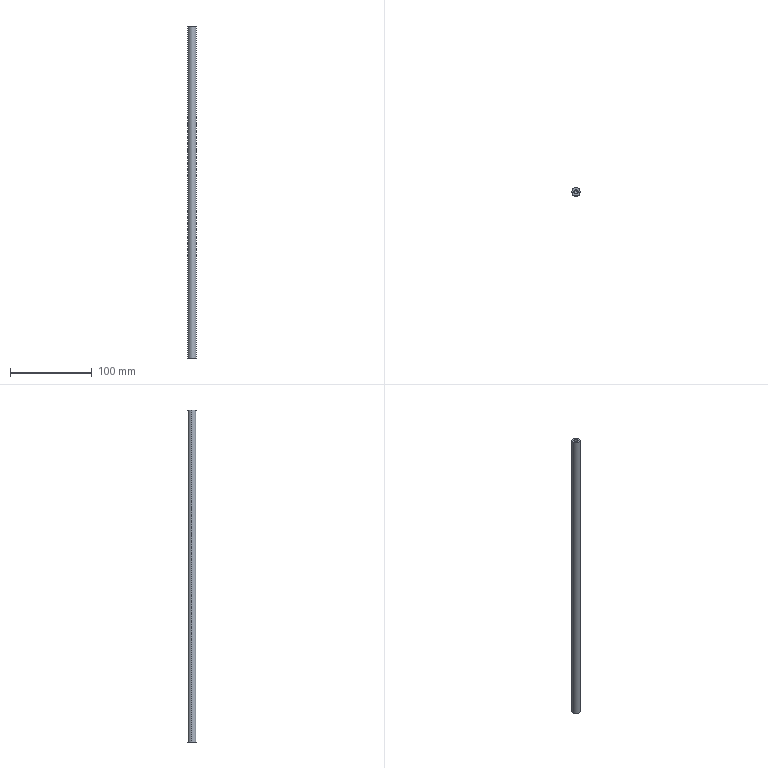Component | SolidWorks | SmoothRod-2 | 1 solid | 16 faces | box 10 x 10 x 405 mm | volume 31407 mm3 | cone 8 | cylinder 6 | plane 2 | commonest cylinder face diameters 4.2 x4 10 x2
build123d program:
from build123d import *


with BuildPart() as part:
    # Sketch1 → Revolve1 (revolve)
    with BuildSketch(Plane(origin=(0, 0, 0), x_dir=(-1, 0, 0), z_dir=(0, 0, -1)), mode=Mode.PRIVATE) as revolve1_sk:
        Polygon((-188.5, 2.1), (-187.238, 0), (187.238, 0), (188.5, 2.1), (202.075, 2.1), (202.5, 2.525), (202.5, 5), (-202.5, 5), (-202.5, 2.525), (-202.075, 2.1), align=None)
    revolve(revolve1_sk.sketch.rotate(Axis((202.5, 0, 0), (-1, 0, 0)), 270), axis=Axis((202.5, 0, 0), (-1, 0, 0)))


solid = part.part

# Placed as in the assembly
solid = solid.moved(Location((210.793, 596, 0), (0, 90, 0)))